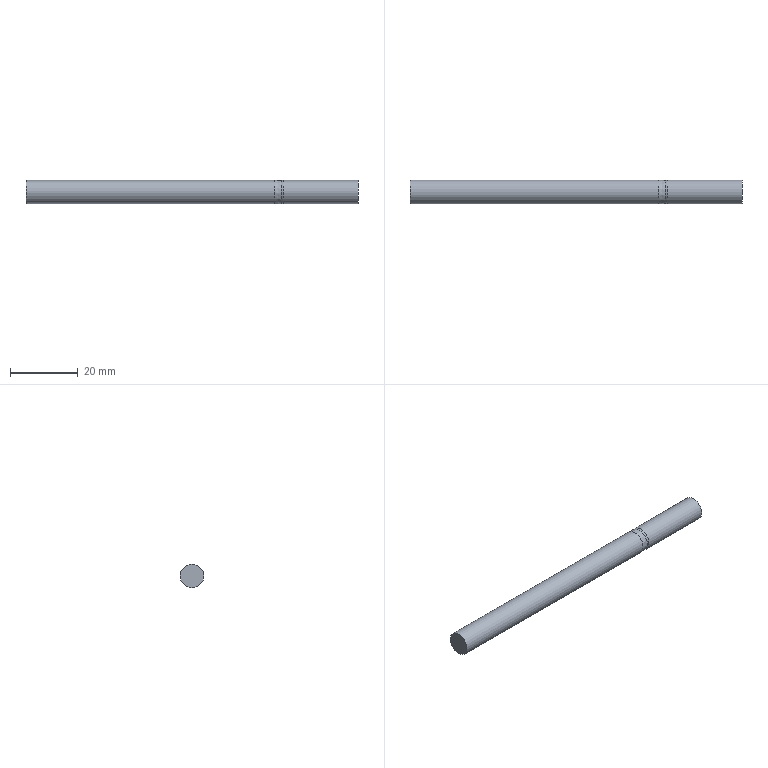Component | NX | SCREW_ROD | 1 solid | 6 faces | box 98 x 6.99 x 6.99 mm | volume 3753 mm3 | plane 2 | cylinder 2 | cone 2 | commonest cylinder face diameters 6.985 x2
STEP:
#1=CARTESIAN_POINT('',(0.,0.,0.));
#2=DIRECTION('',(0.,0.,1.));
#3=DIRECTION('',(1.,0.,0.));
#4=AXIS2_PLACEMENT_3D('',#1,#2,#3);
#5=CARTESIAN_POINT('',(-39.,149.5,-297.993));
#6=VERTEX_POINT('',#5);
#7=CARTESIAN_POINT('',(-39.,149.5,-294.5));
#8=DIRECTION('',(1.,0.,0.));
#9=DIRECTION('',(0.,0.,-1.));
#10=AXIS2_PLACEMENT_3D('',#7,#8,#9);
#11=CIRCLE('',#10,3.493);
#12=CARTESIAN_POINT('',(-39.,149.5,-294.5));
#13=DIRECTION('',(1.,0.,0.));
#14=DIRECTION('',(0.,0.,-1.));
#15=AXIS2_PLACEMENT_3D('',#12,#13,#14);
#16=PLANE('',#15);
#17=CARTESIAN_POINT('',(0.,0.));
#18=DIRECTION('',(1.,0.));
#19=AXIS2_PLACEMENT_2D('',#17,#18);
#20=CIRCLE('',#19,3.493);
#21=(GEOMETRIC_REPRESENTATION_CONTEXT(2)PARAMETRIC_REPRESENTATION_CONTEXT()REPRESENTATION_CONTEXT('',''));
#22=DEFINITIONAL_REPRESENTATION('',(#20),#21);
#23=PCURVE('',#16,#22);
#24=CARTESIAN_POINT('',(-39.,149.5,-294.5));
#25=DIRECTION('',(1.,0.,0.));
#26=DIRECTION('',(0.,0.,-1.));
#27=AXIS2_PLACEMENT_3D('',#24,#25,#26);
#28=CYLINDRICAL_SURFACE('',#27,3.493);
#29=CARTESIAN_POINT('',(0.,0.));
#30=DIRECTION('',(1.,0.));
#31=VECTOR('',#30,1.);
#32=LINE('',#29,#31);
#33=(GEOMETRIC_REPRESENTATION_CONTEXT(2)PARAMETRIC_REPRESENTATION_CONTEXT()REPRESENTATION_CONTEXT('',''));
#34=DEFINITIONAL_REPRESENTATION('',(#32),#33);
#35=PCURVE('',#28,#34);
#36=SURFACE_CURVE('',#11,(#23,#35),.PCURVE_S1.);
#37=EDGE_CURVE('',#6,#6,#36,.T.);
#38=ORIENTED_EDGE('',*,*,#37,.F.);
#39=EDGE_LOOP('',(#38));
#40=FACE_BOUND('',#39,.T.);
#41=ADVANCED_FACE('',(#40),#16,.F.);
#42=CARTESIAN_POINT('',(59.,149.5,-297.993));
#43=VERTEX_POINT('',#42);
#44=CARTESIAN_POINT('',(59.,149.5,-294.5));
#45=DIRECTION('',(1.,0.,0.));
#46=DIRECTION('',(0.,0.,-1.));
#47=AXIS2_PLACEMENT_3D('',#44,#45,#46);
#48=CIRCLE('',#47,3.493);
#49=CARTESIAN_POINT('',(59.,149.5,-294.5));
#50=DIRECTION('',(1.,0.,0.));
#51=DIRECTION('',(0.,0.,-1.));
#52=AXIS2_PLACEMENT_3D('',#49,#50,#51);
#53=PLANE('',#52);
#54=CARTESIAN_POINT('',(0.,0.));
#55=DIRECTION('',(1.,0.));
#56=AXIS2_PLACEMENT_2D('',#54,#55);
#57=CIRCLE('',#56,3.493);
#58=(GEOMETRIC_REPRESENTATION_CONTEXT(2)PARAMETRIC_REPRESENTATION_CONTEXT()REPRESENTATION_CONTEXT('',''));
#59=DEFINITIONAL_REPRESENTATION('',(#57),#58);
#60=PCURVE('',#53,#59);
#61=CARTESIAN_POINT('',(-39.,149.5,-294.5));
#62=DIRECTION('',(1.,0.,0.));
#63=DIRECTION('',(0.,0.,-1.));
#64=AXIS2_PLACEMENT_3D('',#61,#62,#63);
#65=CYLINDRICAL_SURFACE('',#64,3.493);
#66=CARTESIAN_POINT('',(0.,98.));
#67=DIRECTION('',(1.,0.));
#68=VECTOR('',#67,1.);
#69=LINE('',#66,#68);
#70=(GEOMETRIC_REPRESENTATION_CONTEXT(2)PARAMETRIC_REPRESENTATION_CONTEXT()REPRESENTATION_CONTEXT('',''));
#71=DEFINITIONAL_REPRESENTATION('',(#69),#70);
#72=PCURVE('',#65,#71);
#73=SURFACE_CURVE('',#48,(#60,#72),.PCURVE_S1.);
#74=EDGE_CURVE('',#43,#43,#73,.T.);
#75=ORIENTED_EDGE('',*,*,#74,.T.);
#76=EDGE_LOOP('',(#75));
#77=FACE_BOUND('',#76,.T.);
#78=ADVANCED_FACE('',(#77),#53,.T.);
#79=ORIENTED_EDGE('',*,*,#74,.F.);
#80=CARTESIAN_POINT('',(37.,149.5,-297.993));
#81=VERTEX_POINT('',#80);
#82=CARTESIAN_POINT('',(37.,149.5,-297.993));
#83=CARTESIAN_POINT('',(59.,149.5,-297.993));
#84=B_SPLINE_CURVE_WITH_KNOTS('',1,(#82,#83),.UNSPECIFIED.,.F.,.F.,(2,2),(76.,98.),.PIECEWISE_BEZIER_KNOTS.);
#85=CARTESIAN_POINT('',(0.,0.));
#86=DIRECTION('',(0.,1.));
#87=VECTOR('',#86,1.);
#88=LINE('',#85,#87);
#89=(GEOMETRIC_REPRESENTATION_CONTEXT(2)PARAMETRIC_REPRESENTATION_CONTEXT()REPRESENTATION_CONTEXT('',''));
#90=DEFINITIONAL_REPRESENTATION('',(#88),#89);
#91=PCURVE('',#65,#90);
#92=CARTESIAN_POINT('',(6.283,0.));
#93=DIRECTION('',(0.,1.));
#94=VECTOR('',#93,1.);
#95=LINE('',#92,#94);
#96=(GEOMETRIC_REPRESENTATION_CONTEXT(2)PARAMETRIC_REPRESENTATION_CONTEXT()REPRESENTATION_CONTEXT('',''));
#97=DEFINITIONAL_REPRESENTATION('',(#95),#96);
#98=PCURVE('',#65,#97);
#99=SEAM_CURVE('',#84,(#91,#98),.PCURVE_S1.);
#100=EDGE_CURVE('',#81,#43,#99,.T.);
#101=ORIENTED_EDGE('',*,*,#100,.F.);
#102=CARTESIAN_POINT('',(37.,149.5,-294.5));
#103=DIRECTION('',(1.,0.,0.));
#104=DIRECTION('',(0.,0.,-1.));
#105=AXIS2_PLACEMENT_3D('',#102,#103,#104);
#106=CIRCLE('',#105,3.493);
#107=CARTESIAN_POINT('',(0.,76.));
#108=DIRECTION('',(1.,0.));
#109=VECTOR('',#108,1.);
#110=LINE('',#107,#109);
#111=(GEOMETRIC_REPRESENTATION_CONTEXT(2)PARAMETRIC_REPRESENTATION_CONTEXT()REPRESENTATION_CONTEXT('',''));
#112=DEFINITIONAL_REPRESENTATION('',(#110),#111);
#113=PCURVE('',#65,#112);
#114=CARTESIAN_POINT('',(36.375,149.5,-294.5));
#115=DIRECTION('',(1.,0.,0.));
#116=DIRECTION('',(0.,0.,-1.));
#117=AXIS2_PLACEMENT_3D('',#114,#115,#116);
#118=CONICAL_SURFACE('',#117,3.4,0.1468);
#119=CARTESIAN_POINT('',(0.,0.6249));
#120=DIRECTION('',(1.,0.));
#121=VECTOR('',#120,1.);
#122=LINE('',#119,#121);
#123=(GEOMETRIC_REPRESENTATION_CONTEXT(2)PARAMETRIC_REPRESENTATION_CONTEXT()REPRESENTATION_CONTEXT('',''));
#124=DEFINITIONAL_REPRESENTATION('',(#122),#123);
#125=PCURVE('',#118,#124);
#126=SURFACE_CURVE('',#106,(#113,#125),.PCURVE_S1.);
#127=EDGE_CURVE('',#81,#81,#126,.T.);
#128=ORIENTED_EDGE('',*,*,#127,.T.);
#129=ORIENTED_EDGE('',*,*,#100,.T.);
#130=EDGE_LOOP('',(#79,#101,#128,#129));
#131=FACE_BOUND('',#130,.T.);
#132=ADVANCED_FACE('',(#131),#65,.T.);
#133=ORIENTED_EDGE('',*,*,#127,.F.);
#134=CARTESIAN_POINT('',(36.375,149.5,-297.9));
#135=VERTEX_POINT('',#134);
#136=CARTESIAN_POINT('',(36.375,149.5,-297.9));
#137=CARTESIAN_POINT('',(37.,149.5,-297.993));
#138=B_SPLINE_CURVE_WITH_KNOTS('',1,(#136,#137),.UNSPECIFIED.,.F.,.F.,(2,2),(0.,0.6317),.PIECEWISE_BEZIER_KNOTS.);
#139=CARTESIAN_POINT('',(0.,0.));
#140=DIRECTION('',(0.,1.));
#141=VECTOR('',#140,1.);
#142=LINE('',#139,#141);
#143=(GEOMETRIC_REPRESENTATION_CONTEXT(2)PARAMETRIC_REPRESENTATION_CONTEXT()REPRESENTATION_CONTEXT('',''));
#144=DEFINITIONAL_REPRESENTATION('',(#142),#143);
#145=PCURVE('',#118,#144);
#146=CARTESIAN_POINT('',(6.283,0.));
#147=DIRECTION('',(0.,1.));
#148=VECTOR('',#147,1.);
#149=LINE('',#146,#148);
#150=(GEOMETRIC_REPRESENTATION_CONTEXT(2)PARAMETRIC_REPRESENTATION_CONTEXT()REPRESENTATION_CONTEXT('',''));
#151=DEFINITIONAL_REPRESENTATION('',(#149),#150);
#152=PCURVE('',#118,#151);
#153=SEAM_CURVE('',#138,(#145,#152),.PCURVE_S1.);
#154=EDGE_CURVE('',#135,#81,#153,.T.);
#155=ORIENTED_EDGE('',*,*,#154,.F.);
#156=CARTESIAN_POINT('',(36.375,149.5,-294.5));
#157=DIRECTION('',(1.,0.,0.));
#158=DIRECTION('',(0.,0.,-1.));
#159=AXIS2_PLACEMENT_3D('',#156,#157,#158);
#160=CIRCLE('',#159,3.4);
#161=CARTESIAN_POINT('',(0.,0.));
#162=DIRECTION('',(1.,0.));
#163=VECTOR('',#162,1.);
#164=LINE('',#161,#163);
#165=(GEOMETRIC_REPRESENTATION_CONTEXT(2)PARAMETRIC_REPRESENTATION_CONTEXT()REPRESENTATION_CONTEXT('',''));
#166=DEFINITIONAL_REPRESENTATION('',(#164),#165);
#167=PCURVE('',#118,#166);
#168=CARTESIAN_POINT('',(34.5,149.5,-294.5));
#169=DIRECTION('',(-1.,0.,0.));
#170=DIRECTION('',(0.,0.,1.));
#171=AXIS2_PLACEMENT_3D('',#168,#169,#170);
#172=CONICAL_SURFACE('',#171,3.493,0.04925);
#173=CARTESIAN_POINT('',(9.425,-1.875));
#174=DIRECTION('',(-1.,0.));
#175=VECTOR('',#174,1.);
#176=LINE('',#173,#175);
#177=(GEOMETRIC_REPRESENTATION_CONTEXT(2)PARAMETRIC_REPRESENTATION_CONTEXT()REPRESENTATION_CONTEXT('',''));
#178=DEFINITIONAL_REPRESENTATION('',(#176),#177);
#179=PCURVE('',#172,#178);
#180=SURFACE_CURVE('',#160,(#167,#179),.PCURVE_S1.);
#181=EDGE_CURVE('',#135,#135,#180,.T.);
#182=ORIENTED_EDGE('',*,*,#181,.T.);
#183=ORIENTED_EDGE('',*,*,#154,.T.);
#184=EDGE_LOOP('',(#133,#155,#182,#183));
#185=FACE_BOUND('',#184,.T.);
#186=ADVANCED_FACE('',(#185),#118,.T.);
#187=ORIENTED_EDGE('',*,*,#181,.F.);
#188=CARTESIAN_POINT('',(34.5,149.5,-297.993));
#189=VERTEX_POINT('',#188);
#190=CARTESIAN_POINT('',(36.375,149.5,-297.9));
#191=CARTESIAN_POINT('',(34.5,149.5,-297.993));
#192=B_SPLINE_CURVE_WITH_KNOTS('',1,(#190,#191),.UNSPECIFIED.,.F.,.F.,(2,2),(-1.877,-0.),.PIECEWISE_BEZIER_KNOTS.);
#193=CARTESIAN_POINT('',(9.425,0.));
#194=DIRECTION('',(0.,1.));
#195=VECTOR('',#194,1.);
#196=LINE('',#193,#195);
#197=(GEOMETRIC_REPRESENTATION_CONTEXT(2)PARAMETRIC_REPRESENTATION_CONTEXT()REPRESENTATION_CONTEXT('',''));
#198=DEFINITIONAL_REPRESENTATION('',(#196),#197);
#199=PCURVE('',#172,#198);
#200=CARTESIAN_POINT('',(3.142,0.));
#201=DIRECTION('',(0.,1.));
#202=VECTOR('',#201,1.);
#203=LINE('',#200,#202);
#204=(GEOMETRIC_REPRESENTATION_CONTEXT(2)PARAMETRIC_REPRESENTATION_CONTEXT()REPRESENTATION_CONTEXT('',''));
#205=DEFINITIONAL_REPRESENTATION('',(#203),#204);
#206=PCURVE('',#172,#205);
#207=SEAM_CURVE('',#192,(#199,#206),.PCURVE_S1.);
#208=EDGE_CURVE('',#135,#189,#207,.T.);
#209=ORIENTED_EDGE('',*,*,#208,.T.);
#210=CARTESIAN_POINT('',(34.5,149.5,-294.5));
#211=DIRECTION('',(1.,0.,0.));
#212=DIRECTION('',(0.,0.,-1.));
#213=AXIS2_PLACEMENT_3D('',#210,#211,#212);
#214=CIRCLE('',#213,3.493);
#215=CARTESIAN_POINT('',(9.425,-0.));
#216=DIRECTION('',(-1.,0.));
#217=VECTOR('',#216,1.);
#218=LINE('',#215,#217);
#219=(GEOMETRIC_REPRESENTATION_CONTEXT(2)PARAMETRIC_REPRESENTATION_CONTEXT()REPRESENTATION_CONTEXT('',''));
#220=DEFINITIONAL_REPRESENTATION('',(#218),#219);
#221=PCURVE('',#172,#220);
#222=CARTESIAN_POINT('',(0.,73.5));
#223=DIRECTION('',(1.,0.));
#224=VECTOR('',#223,1.);
#225=LINE('',#222,#224);
#226=(GEOMETRIC_REPRESENTATION_CONTEXT(2)PARAMETRIC_REPRESENTATION_CONTEXT()REPRESENTATION_CONTEXT('',''));
#227=DEFINITIONAL_REPRESENTATION('',(#225),#226);
#228=PCURVE('',#28,#227);
#229=SURFACE_CURVE('',#214,(#221,#228),.PCURVE_S1.);
#230=EDGE_CURVE('',#189,#189,#229,.T.);
#231=ORIENTED_EDGE('',*,*,#230,.T.);
#232=ORIENTED_EDGE('',*,*,#208,.F.);
#233=EDGE_LOOP('',(#187,#209,#231,#232));
#234=FACE_BOUND('',#233,.T.);
#235=ADVANCED_FACE('',(#234),#172,.T.);
#236=ORIENTED_EDGE('',*,*,#230,.F.);
#237=CARTESIAN_POINT('',(-39.,149.5,-297.993));
#238=CARTESIAN_POINT('',(34.5,149.5,-297.993));
#239=B_SPLINE_CURVE_WITH_KNOTS('',1,(#237,#238),.UNSPECIFIED.,.F.,.F.,(2,2),(0.,73.5),.PIECEWISE_BEZIER_KNOTS.);
#240=CARTESIAN_POINT('',(0.,0.));
#241=DIRECTION('',(0.,1.));
#242=VECTOR('',#241,1.);
#243=LINE('',#240,#242);
#244=(GEOMETRIC_REPRESENTATION_CONTEXT(2)PARAMETRIC_REPRESENTATION_CONTEXT()REPRESENTATION_CONTEXT('',''));
#245=DEFINITIONAL_REPRESENTATION('',(#243),#244);
#246=PCURVE('',#28,#245);
#247=CARTESIAN_POINT('',(6.283,0.));
#248=DIRECTION('',(0.,1.));
#249=VECTOR('',#248,1.);
#250=LINE('',#247,#249);
#251=(GEOMETRIC_REPRESENTATION_CONTEXT(2)PARAMETRIC_REPRESENTATION_CONTEXT()REPRESENTATION_CONTEXT('',''));
#252=DEFINITIONAL_REPRESENTATION('',(#250),#251);
#253=PCURVE('',#28,#252);
#254=SEAM_CURVE('',#239,(#246,#253),.PCURVE_S1.);
#255=EDGE_CURVE('',#6,#189,#254,.T.);
#256=ORIENTED_EDGE('',*,*,#255,.F.);
#257=ORIENTED_EDGE('',*,*,#37,.T.);
#258=ORIENTED_EDGE('',*,*,#255,.T.);
#259=EDGE_LOOP('',(#236,#256,#257,#258));
#260=FACE_BOUND('',#259,.T.);
#261=ADVANCED_FACE('',(#260),#28,.T.);
#262=CLOSED_SHELL('',(#41,#78,#132,#186,#235,#261));
#263=MANIFOLD_SOLID_BREP('',#262);
#264=(LENGTH_UNIT()NAMED_UNIT(*)SI_UNIT(.MILLI.,.METRE.));
#265=UNCERTAINTY_MEASURE_WITH_UNIT(LENGTH_MEASURE(0.00001),#264,'','');
#266=(NAMED_UNIT(*)PLANE_ANGLE_UNIT()SI_UNIT($,.RADIAN.));
#267=(NAMED_UNIT(*)SI_UNIT($,.STERADIAN.)SOLID_ANGLE_UNIT());
#268=(GEOMETRIC_REPRESENTATION_CONTEXT(3)GLOBAL_UNCERTAINTY_ASSIGNED_CONTEXT((#265))GLOBAL_UNIT_ASSIGNED_CONTEXT((#264,#266,#267))REPRESENTATION_CONTEXT('',''));
#269=ADVANCED_BREP_SHAPE_REPRESENTATION('',(#4,#263),#268);